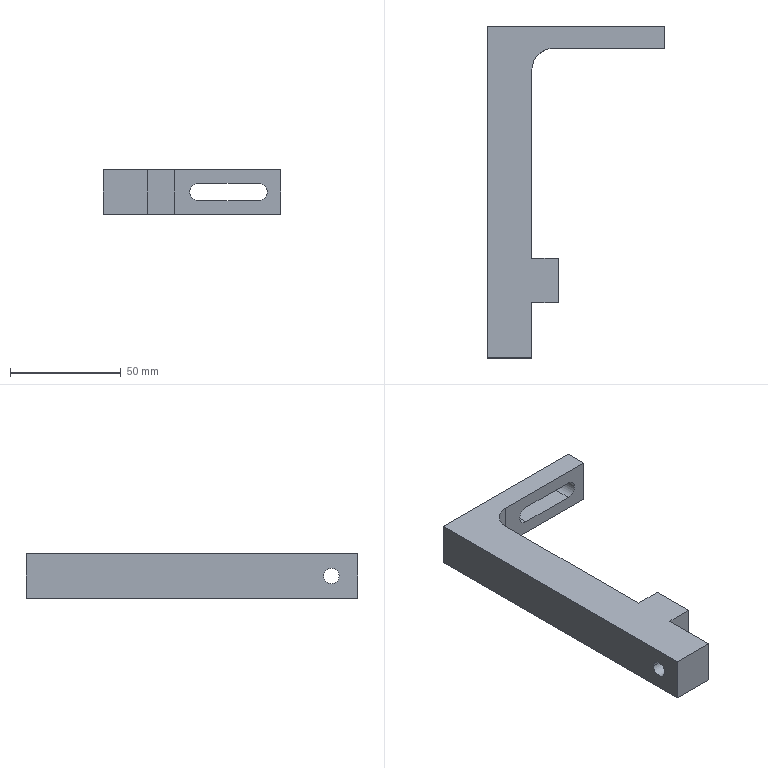Component | SolidWorks | GuideMechanism-1_LimitRollerSeat-1 | 1 solid | 19 faces | box 80 x 150 x 20 mm | volume 73797 mm3 | plane 14 | cylinder 5 | commonest cylinder face diameters 7 x2 8 x2 20 x1
build123d program:
from build123d import *

# Parameters (mm, degrees)
SKETCH1_W           = 80
SKETCH1_H           = 125
BOSS_EXTRUDE1_DEPTH = 20
SKETCH2_W           = 60
SKETCH2_H           = 95
CUT_EXTRUDE1_DEPTH  = 77.852
BOSS_EXTRUDE2_DEPTH = 20
SKETCH4_R           = 4
CUT_EXTRUDE2_DEPTH  = 157.525
CUT_EXTRUDE3_DEPTH  = 157.525
SKETCH6_R           = 3.5
CUT_EXTRUDE4_DEPTH  = 121.234
SKETCH7_W           = 48
SKETCH7_H           = 20
CUT_EXTRUDE5_DEPTH  = 99.266
FILLET1_R           = 10


with BuildPart() as part:
    # Sketch1 → Boss-Extrude1 (new body)
    with BuildSketch(Plane.XY):
        Rectangle(SKETCH1_W, SKETCH1_H)
    extrude(amount=BOSS_EXTRUDE1_DEPTH)

    # Sketch2 → Cut-Extrude1 (cut, through all)
    with BuildSketch(Plane.XY.offset(20)):
        with Locations((10, 5)):
            Rectangle(SKETCH2_W, SKETCH2_H)
    extrude(amount=-CUT_EXTRUDE1_DEPTH, mode=Mode.SUBTRACT)

    # Sketch3 → Boss-Extrude2 (add)
    with BuildSketch(Plane.XY.offset(20)):
        Polygon((-20, -42.5), (-20, -87.5), (-40, -87.5), (-40, -62.5), align=None)
    extrude(amount=-BOSS_EXTRUDE2_DEPTH)

    # Sketch4 → Cut-Extrude2 (cut, through all)
    with BuildSketch(Plane(origin=(0, 62.5, 0), x_dir=(1, 0, 0), z_dir=(0, 1, 0))):
        with Locations(Location((30, -10, 0), (0, 0, 270))):
            Circle(SKETCH4_R)
    extrude(amount=-CUT_EXTRUDE2_DEPTH, mode=Mode.SUBTRACT)

    # Sketch5 → Cut-Extrude3 (cut, through all)
    with BuildSketch(Plane(origin=(0, 62.5, 0), x_dir=(1, 0, 0), z_dir=(0, 1, 0))):
        with BuildLine():
            Line((30, -14), (3, -14))
            ThreePointArc((3, -14), (-1, -10), (3, -6))
            Line((3, -6), (30, -6))
            ThreePointArc((30, -6), (34, -10), (30, -14))
        make_face()
    extrude(amount=-CUT_EXTRUDE3_DEPTH, mode=Mode.SUBTRACT)

    # Sketch6 → Cut-Extrude4 (cut, through all)
    with BuildSketch(Plane.ZY.offset(40)):
        with Locations(Location((10, -75.5, 0), (0, 0, 270))):
            Circle(SKETCH6_R)
    extrude(amount=-CUT_EXTRUDE4_DEPTH, mode=Mode.SUBTRACT)

    # Sketch7 → Cut-Extrude5 (cut, through all)
    with BuildSketch(Plane.XY.offset(20)):
        with Locations((16, -52.5)):
            Rectangle(SKETCH7_W, SKETCH7_H)
    extrude(amount=-CUT_EXTRUDE5_DEPTH, mode=Mode.SUBTRACT)

    # Fillet1
    fillet1_edges = [part.edges().sort_by_distance(p)[0] for p in [
        (-20, 52.5, 10),
    ]]
    fillet(fillet1_edges, radius=FILLET1_R)


solid = part.part

# Placed as in the assembly
solid = solid.moved(Location((-505.272, -306.266, 1151.5), (0, 0, 0)))
STEP:
#1=COLOUR_RGB('',0.7922,0.8196,0.9333);
#2=FILL_AREA_STYLE_COLOUR('',#1);
#3=FILL_AREA_STYLE('',(#2));
#4=SURFACE_STYLE_FILL_AREA(#3);
#5=SURFACE_SIDE_STYLE('',(#4));
#6=SURFACE_STYLE_USAGE(.BOTH.,#5);
#7=PRESENTATION_STYLE_ASSIGNMENT((#6));
#8=CARTESIAN_POINT('',(-20.68,-15.168,45.728));
#9=VERTEX_POINT('',#8);
#10=CARTESIAN_POINT('',(-20.68,-14.892,45.728));
#11=VERTEX_POINT('',#10);
#12=CARTESIAN_POINT('',(-20.68,-15.03,45.728));
#13=DIRECTION('',(1.,0.,0.));
#14=DIRECTION('',(0.,1.,0.));
#15=AXIS2_PLACEMENT_3D('',#12,#13,#14);
#16=CIRCLE('',#15,0.1378);
#17=EDGE_CURVE('',#9,#11,#16,.T.);
#18=ORIENTED_EDGE('',*,*,#17,.T.);
#19=CARTESIAN_POINT('',(-21.467,-14.892,45.728));
#20=VERTEX_POINT('',#19);
#21=CARTESIAN_POINT('',(-18.318,-14.892,45.728));
#22=DIRECTION('',(-1.,-0.,0.));
#23=VECTOR('',#22,39.37);
#24=LINE('',#21,#23);
#25=EDGE_CURVE('',#11,#20,#24,.T.);
#26=ORIENTED_EDGE('',*,*,#25,.T.);
#27=CARTESIAN_POINT('',(-21.467,-15.168,45.728));
#28=VERTEX_POINT('',#27);
#29=CARTESIAN_POINT('',(-21.467,-15.03,45.728));
#30=DIRECTION('',(-1.,-0.,0.));
#31=DIRECTION('',(0.,-1.,0.));
#32=AXIS2_PLACEMENT_3D('',#29,#30,#31);
#33=CIRCLE('',#32,0.1378);
#34=EDGE_CURVE('',#20,#28,#33,.T.);
#35=ORIENTED_EDGE('',*,*,#34,.T.);
#36=CARTESIAN_POINT('',(-18.318,-15.168,45.728));
#37=DIRECTION('',(-1.,-0.,0.));
#38=VECTOR('',#37,39.37);
#39=LINE('',#36,#38);
#40=EDGE_CURVE('',#9,#28,#39,.T.);
#41=ORIENTED_EDGE('',*,*,#40,.F.);
#42=EDGE_LOOP('',(#18,#26,#35,#41));
#43=FACE_OUTER_BOUND('',#42,.T.);
#44=CARTESIAN_POINT('',(-18.318,-15.03,45.728));
#45=DIRECTION('',(-1.,-0.,0.));
#46=DIRECTION('',(0.,-1.,0.));
#47=AXIS2_PLACEMENT_3D('',#44,#45,#46);
#48=CYLINDRICAL_SURFACE('',#47,0.1378);
#49=ADVANCED_FACE('',(#43),#48,.F.);
#50=CARTESIAN_POINT('',(-18.711,-9.991,45.886));
#51=VERTEX_POINT('',#50);
#52=CARTESIAN_POINT('',(-18.711,-9.597,45.886));
#53=VERTEX_POINT('',#52);
#54=CARTESIAN_POINT('',(-18.711,-15.503,45.886));
#55=DIRECTION('',(0.,1.,0.));
#56=VECTOR('',#55,39.37);
#57=LINE('',#54,#56);
#58=EDGE_CURVE('',#51,#53,#57,.T.);
#59=ORIENTED_EDGE('',*,*,#58,.T.);
#60=CARTESIAN_POINT('',(-18.711,-9.597,45.571));
#61=VERTEX_POINT('',#60);
#62=CARTESIAN_POINT('',(-18.711,-9.597,45.728));
#63=DIRECTION('',(0.,1.,0.));
#64=DIRECTION('',(0.,0.,1.));
#65=AXIS2_PLACEMENT_3D('',#62,#63,#64);
#66=CIRCLE('',#65,0.1575);
#67=EDGE_CURVE('',#53,#61,#66,.T.);
#68=ORIENTED_EDGE('',*,*,#67,.T.);
#69=CARTESIAN_POINT('',(-18.711,-9.991,45.571));
#70=VERTEX_POINT('',#69);
#71=CARTESIAN_POINT('',(-18.711,-15.503,45.571));
#72=DIRECTION('',(0.,1.,0.));
#73=VECTOR('',#72,39.37);
#74=LINE('',#71,#73);
#75=EDGE_CURVE('',#70,#61,#74,.T.);
#76=ORIENTED_EDGE('',*,*,#75,.F.);
#77=CARTESIAN_POINT('',(-18.711,-9.991,45.728));
#78=DIRECTION('',(0.,1.,0.));
#79=DIRECTION('',(0.,0.,1.));
#80=AXIS2_PLACEMENT_3D('',#77,#78,#79);
#81=CIRCLE('',#80,0.1575);
#82=EDGE_CURVE('',#51,#70,#81,.T.);
#83=ORIENTED_EDGE('',*,*,#82,.F.);
#84=EDGE_LOOP('',(#59,#68,#76,#83));
#85=FACE_OUTER_BOUND('',#84,.T.);
#86=CARTESIAN_POINT('',(-18.711,-15.503,45.728));
#87=DIRECTION('',(0.,1.,0.));
#88=DIRECTION('',(0.,0.,1.));
#89=AXIS2_PLACEMENT_3D('',#86,#87,#88);
#90=CYLINDRICAL_SURFACE('',#89,0.1575);
#91=ADVANCED_FACE('',(#85),#90,.F.);
#92=CARTESIAN_POINT('',(-18.318,-9.991,46.122));
#93=VERTEX_POINT('',#92);
#94=CARTESIAN_POINT('',(-18.318,-9.597,46.122));
#95=VERTEX_POINT('',#94);
#96=CARTESIAN_POINT('',(-18.318,-9.597,46.122));
#97=DIRECTION('',(-0.,1.,0.));
#98=VECTOR('',#97,39.37);
#99=LINE('',#96,#98);
#100=EDGE_CURVE('',#93,#95,#99,.T.);
#101=ORIENTED_EDGE('',*,*,#100,.F.);
#102=CARTESIAN_POINT('',(-18.318,-9.991,45.335));
#103=VERTEX_POINT('',#102);
#104=CARTESIAN_POINT('',(-18.318,-9.991,45.335));
#105=DIRECTION('',(0.,0.,1.));
#106=VECTOR('',#105,39.37);
#107=LINE('',#104,#106);
#108=EDGE_CURVE('',#103,#93,#107,.T.);
#109=ORIENTED_EDGE('',*,*,#108,.F.);
#110=CARTESIAN_POINT('',(-18.318,-9.597,45.335));
#111=VERTEX_POINT('',#110);
#112=CARTESIAN_POINT('',(-18.318,-9.597,45.335));
#113=DIRECTION('',(-0.,1.,0.));
#114=VECTOR('',#113,39.37);
#115=LINE('',#112,#114);
#116=EDGE_CURVE('',#103,#111,#115,.T.);
#117=ORIENTED_EDGE('',*,*,#116,.T.);
#118=CARTESIAN_POINT('',(-18.318,-9.597,46.122));
#119=DIRECTION('',(0.,0.,-1.));
#120=VECTOR('',#119,39.37);
#121=LINE('',#118,#120);
#122=EDGE_CURVE('',#95,#111,#121,.T.);
#123=ORIENTED_EDGE('',*,*,#122,.F.);
#124=EDGE_LOOP('',(#101,#109,#117,#123));
#125=FACE_OUTER_BOUND('',#124,.T.);
#126=CARTESIAN_POINT('',(-18.318,-9.597,46.122));
#127=DIRECTION('',(-1.,-0.,0.));
#128=DIRECTION('',(0.,-1.,0.));
#129=AXIS2_PLACEMENT_3D('',#126,#127,#128);
#130=PLANE('',#129);
#131=ADVANCED_FACE('',(#125),#130,.F.);
#132=ORIENTED_EDGE('',*,*,#67,.F.);
#133=CARTESIAN_POINT('',(-19.774,-9.597,45.886));
#134=VERTEX_POINT('',#133);
#135=CARTESIAN_POINT('',(-18.711,-9.597,45.886));
#136=DIRECTION('',(1.,0.,-0.));
#137=VECTOR('',#136,39.37);
#138=LINE('',#135,#137);
#139=EDGE_CURVE('',#134,#53,#138,.T.);
#140=ORIENTED_EDGE('',*,*,#139,.F.);
#141=CARTESIAN_POINT('',(-19.774,-9.597,45.571));
#142=VERTEX_POINT('',#141);
#143=CARTESIAN_POINT('',(-19.774,-9.597,45.728));
#144=DIRECTION('',(0.,1.,0.));
#145=DIRECTION('',(0.,0.,1.));
#146=AXIS2_PLACEMENT_3D('',#143,#144,#145);
#147=CIRCLE('',#146,0.1575);
#148=EDGE_CURVE('',#142,#134,#147,.T.);
#149=ORIENTED_EDGE('',*,*,#148,.F.);
#150=CARTESIAN_POINT('',(-18.711,-9.597,45.571));
#151=DIRECTION('',(-1.,0.,0.));
#152=VECTOR('',#151,39.37);
#153=LINE('',#150,#152);
#154=EDGE_CURVE('',#61,#142,#153,.T.);
#155=ORIENTED_EDGE('',*,*,#154,.F.);
#156=EDGE_LOOP('',(#132,#140,#149,#155));
#157=FACE_BOUND('',#156,.T.);
#158=CARTESIAN_POINT('',(-21.467,-9.597,45.335));
#159=VERTEX_POINT('',#158);
#160=CARTESIAN_POINT('',(-21.467,-9.597,45.335));
#161=DIRECTION('',(-1.,0.,0.));
#162=VECTOR('',#161,39.37);
#163=LINE('',#160,#162);
#164=EDGE_CURVE('',#111,#159,#163,.T.);
#165=ORIENTED_EDGE('',*,*,#164,.T.);
#166=CARTESIAN_POINT('',(-21.467,-9.597,46.122));
#167=VERTEX_POINT('',#166);
#168=CARTESIAN_POINT('',(-21.467,-9.597,46.122));
#169=DIRECTION('',(0.,0.,-1.));
#170=VECTOR('',#169,39.37);
#171=LINE('',#168,#170);
#172=EDGE_CURVE('',#167,#159,#171,.T.);
#173=ORIENTED_EDGE('',*,*,#172,.F.);
#174=CARTESIAN_POINT('',(-21.467,-9.597,46.122));
#175=DIRECTION('',(-1.,0.,0.));
#176=VECTOR('',#175,39.37);
#177=LINE('',#174,#176);
#178=EDGE_CURVE('',#95,#167,#177,.T.);
#179=ORIENTED_EDGE('',*,*,#178,.F.);
#180=ORIENTED_EDGE('',*,*,#122,.T.);
#181=EDGE_LOOP('',(#165,#173,#179,#180));
#182=FACE_OUTER_BOUND('',#181,.T.);
#183=CARTESIAN_POINT('',(-21.467,-9.597,46.122));
#184=DIRECTION('',(0.,-1.,0.));
#185=DIRECTION('',(0.,0.,-1.));
#186=AXIS2_PLACEMENT_3D('',#183,#184,#185);
#187=PLANE('',#186);
#188=ADVANCED_FACE('',(#157,#182),#187,.F.);
#189=CARTESIAN_POINT('',(-21.467,-15.03,45.728));
#190=DIRECTION('',(-1.,-0.,0.));
#191=DIRECTION('',(0.,-1.,0.));
#192=AXIS2_PLACEMENT_3D('',#189,#190,#191);
#193=CIRCLE('',#192,0.1378);
#194=EDGE_CURVE('',#28,#20,#193,.T.);
#195=ORIENTED_EDGE('',*,*,#194,.F.);
#196=ORIENTED_EDGE('',*,*,#34,.F.);
#197=EDGE_LOOP('',(#195,#196));
#198=FACE_BOUND('',#197,.T.);
#199=CARTESIAN_POINT('',(-21.467,-15.503,45.335));
#200=VERTEX_POINT('',#199);
#201=CARTESIAN_POINT('',(-21.467,-9.597,45.335));
#202=DIRECTION('',(0.,-1.,0.));
#203=VECTOR('',#202,39.37);
#204=LINE('',#201,#203);
#205=EDGE_CURVE('',#159,#200,#204,.T.);
#206=ORIENTED_EDGE('',*,*,#205,.T.);
#207=CARTESIAN_POINT('',(-21.467,-15.503,46.122));
#208=VERTEX_POINT('',#207);
#209=CARTESIAN_POINT('',(-21.467,-15.503,45.335));
#210=DIRECTION('',(0.,0.,1.));
#211=VECTOR('',#210,39.37);
#212=LINE('',#209,#211);
#213=EDGE_CURVE('',#200,#208,#212,.T.);
#214=ORIENTED_EDGE('',*,*,#213,.T.);
#215=CARTESIAN_POINT('',(-21.467,-9.597,46.122));
#216=DIRECTION('',(0.,-1.,0.));
#217=VECTOR('',#216,39.37);
#218=LINE('',#215,#217);
#219=EDGE_CURVE('',#167,#208,#218,.T.);
#220=ORIENTED_EDGE('',*,*,#219,.F.);
#221=ORIENTED_EDGE('',*,*,#172,.T.);
#222=EDGE_LOOP('',(#206,#214,#220,#221));
#223=FACE_OUTER_BOUND('',#222,.T.);
#224=CARTESIAN_POINT('',(-21.467,-9.597,46.122));
#225=DIRECTION('',(1.,0.,0.));
#226=DIRECTION('',(-0.,1.,0.));
#227=AXIS2_PLACEMENT_3D('',#224,#225,#226);
#228=PLANE('',#227);
#229=ADVANCED_FACE('',(#198,#223),#228,.F.);
#230=CARTESIAN_POINT('',(-20.68,-14.518,45.335));
#231=VERTEX_POINT('',#230);
#232=CARTESIAN_POINT('',(-20.208,-14.518,45.335));
#233=VERTEX_POINT('',#232);
#234=CARTESIAN_POINT('',(-21.467,-14.518,45.335));
#235=DIRECTION('',(1.,0.,0.));
#236=VECTOR('',#235,39.37);
#237=LINE('',#234,#236);
#238=EDGE_CURVE('',#231,#233,#237,.T.);
#239=ORIENTED_EDGE('',*,*,#238,.T.);
#240=CARTESIAN_POINT('',(-20.208,-14.518,46.122));
#241=VERTEX_POINT('',#240);
#242=CARTESIAN_POINT('',(-20.208,-14.518,45.335));
#243=DIRECTION('',(0.,0.,1.));
#244=VECTOR('',#243,39.37);
#245=LINE('',#242,#244);
#246=EDGE_CURVE('',#233,#241,#245,.T.);
#247=ORIENTED_EDGE('',*,*,#246,.T.);
#248=CARTESIAN_POINT('',(-20.68,-14.518,46.122));
#249=VERTEX_POINT('',#248);
#250=CARTESIAN_POINT('',(-21.467,-14.518,46.122));
#251=DIRECTION('',(1.,0.,0.));
#252=VECTOR('',#251,39.37);
#253=LINE('',#250,#252);
#254=EDGE_CURVE('',#249,#241,#253,.T.);
#255=ORIENTED_EDGE('',*,*,#254,.F.);
#256=CARTESIAN_POINT('',(-20.68,-14.518,46.122));
#257=DIRECTION('',(0.,0.,-1.));
#258=VECTOR('',#257,39.37);
#259=LINE('',#256,#258);
#260=EDGE_CURVE('',#249,#231,#259,.T.);
#261=ORIENTED_EDGE('',*,*,#260,.T.);
#262=EDGE_LOOP('',(#239,#247,#255,#261));
#263=FACE_OUTER_BOUND('',#262,.T.);
#264=CARTESIAN_POINT('',(-21.467,-14.518,46.122));
#265=DIRECTION('',(0.,1.,0.));
#266=DIRECTION('',(0.,0.,1.));
#267=AXIS2_PLACEMENT_3D('',#264,#265,#266);
#268=PLANE('',#267);
#269=ADVANCED_FACE('',(#263),#268,.F.);
#270=CARTESIAN_POINT('',(-20.208,-13.731,46.122));
#271=VERTEX_POINT('',#270);
#272=CARTESIAN_POINT('',(-20.208,-13.731,46.122));
#273=DIRECTION('',(0.,-1.,0.));
#274=VECTOR('',#273,39.37);
#275=LINE('',#272,#274);
#276=EDGE_CURVE('',#271,#241,#275,.T.);
#277=ORIENTED_EDGE('',*,*,#276,.F.);
#278=CARTESIAN_POINT('',(-20.68,-13.731,46.122));
#279=VERTEX_POINT('',#278);
#280=CARTESIAN_POINT('',(-18.318,-13.731,46.122));
#281=DIRECTION('',(1.,0.,0.));
#282=VECTOR('',#281,39.37);
#283=LINE('',#280,#282);
#284=EDGE_CURVE('',#279,#271,#283,.T.);
#285=ORIENTED_EDGE('',*,*,#284,.F.);
#286=CARTESIAN_POINT('',(-20.68,-10.384,46.122));
#287=VERTEX_POINT('',#286);
#288=CARTESIAN_POINT('',(-20.68,-9.991,46.122));
#289=DIRECTION('',(0.,-1.,0.));
#290=VECTOR('',#289,39.37);
#291=LINE('',#288,#290);
#292=EDGE_CURVE('',#287,#279,#291,.T.);
#293=ORIENTED_EDGE('',*,*,#292,.F.);
#294=CARTESIAN_POINT('',(-20.286,-9.991,46.122));
#295=VERTEX_POINT('',#294);
#296=CARTESIAN_POINT('',(-20.286,-10.384,46.122));
#297=DIRECTION('',(0.,0.,-1.));
#298=DIRECTION('',(1.,0.,0.));
#299=AXIS2_PLACEMENT_3D('',#296,#297,#298);
#300=CIRCLE('',#299,0.3937);
#301=EDGE_CURVE('',#287,#295,#300,.T.);
#302=ORIENTED_EDGE('',*,*,#301,.T.);
#303=CARTESIAN_POINT('',(-18.318,-9.991,46.122));
#304=DIRECTION('',(-1.,0.,0.));
#305=VECTOR('',#304,39.37);
#306=LINE('',#303,#305);
#307=EDGE_CURVE('',#93,#295,#306,.T.);
#308=ORIENTED_EDGE('',*,*,#307,.F.);
#309=ORIENTED_EDGE('',*,*,#100,.T.);
#310=ORIENTED_EDGE('',*,*,#178,.T.);
#311=ORIENTED_EDGE('',*,*,#219,.T.);
#312=CARTESIAN_POINT('',(-20.68,-15.503,46.122));
#313=VERTEX_POINT('',#312);
#314=CARTESIAN_POINT('',(-20.68,-15.503,46.122));
#315=DIRECTION('',(1.,0.,0.));
#316=VECTOR('',#315,39.37);
#317=LINE('',#314,#316);
#318=EDGE_CURVE('',#208,#313,#317,.T.);
#319=ORIENTED_EDGE('',*,*,#318,.T.);
#320=CARTESIAN_POINT('',(-20.68,-13.731,46.122));
#321=DIRECTION('',(-0.,1.,0.));
#322=VECTOR('',#321,39.37);
#323=LINE('',#320,#322);
#324=EDGE_CURVE('',#313,#249,#323,.T.);
#325=ORIENTED_EDGE('',*,*,#324,.T.);
#326=ORIENTED_EDGE('',*,*,#254,.T.);
#327=EDGE_LOOP('',(#277,#285,#293,#302,#308,#309,#310,#311,#319,#325,#326));
#328=FACE_OUTER_BOUND('',#327,.T.);
#329=CARTESIAN_POINT('',(-19.893,-12.058,46.122));
#330=DIRECTION('',(0.,0.,1.));
#331=DIRECTION('',(1.,0.,0.));
#332=AXIS2_PLACEMENT_3D('',#329,#330,#331);
#333=PLANE('',#332);
#334=ADVANCED_FACE('',(#328),#333,.T.);
#335=CARTESIAN_POINT('',(-20.68,-13.731,45.335));
#336=VERTEX_POINT('',#335);
#337=CARTESIAN_POINT('',(-20.208,-13.731,45.335));
#338=VERTEX_POINT('',#337);
#339=CARTESIAN_POINT('',(-18.318,-13.731,45.335));
#340=DIRECTION('',(1.,0.,0.));
#341=VECTOR('',#340,39.37);
#342=LINE('',#339,#341);
#343=EDGE_CURVE('',#336,#338,#342,.T.);
#344=ORIENTED_EDGE('',*,*,#343,.T.);
#345=CARTESIAN_POINT('',(-20.208,-13.731,45.335));
#346=DIRECTION('',(0.,-1.,0.));
#347=VECTOR('',#346,39.37);
#348=LINE('',#345,#347);
#349=EDGE_CURVE('',#338,#233,#348,.T.);
#350=ORIENTED_EDGE('',*,*,#349,.T.);
#351=ORIENTED_EDGE('',*,*,#238,.F.);
#352=CARTESIAN_POINT('',(-20.68,-15.503,45.335));
#353=VERTEX_POINT('',#352);
#354=CARTESIAN_POINT('',(-20.68,-13.731,45.335));
#355=DIRECTION('',(-0.,1.,0.));
#356=VECTOR('',#355,39.37);
#357=LINE('',#354,#356);
#358=EDGE_CURVE('',#353,#231,#357,.T.);
#359=ORIENTED_EDGE('',*,*,#358,.F.);
#360=CARTESIAN_POINT('',(-20.68,-15.503,45.335));
#361=DIRECTION('',(1.,0.,0.));
#362=VECTOR('',#361,39.37);
#363=LINE('',#360,#362);
#364=EDGE_CURVE('',#200,#353,#363,.T.);
#365=ORIENTED_EDGE('',*,*,#364,.F.);
#366=ORIENTED_EDGE('',*,*,#205,.F.);
#367=ORIENTED_EDGE('',*,*,#164,.F.);
#368=ORIENTED_EDGE('',*,*,#116,.F.);
#369=CARTESIAN_POINT('',(-20.286,-9.991,45.335));
#370=VERTEX_POINT('',#369);
#371=CARTESIAN_POINT('',(-18.318,-9.991,45.335));
#372=DIRECTION('',(-1.,0.,0.));
#373=VECTOR('',#372,39.37);
#374=LINE('',#371,#373);
#375=EDGE_CURVE('',#103,#370,#374,.T.);
#376=ORIENTED_EDGE('',*,*,#375,.T.);
#377=CARTESIAN_POINT('',(-20.68,-10.384,45.335));
#378=VERTEX_POINT('',#377);
#379=CARTESIAN_POINT('',(-20.286,-10.384,45.335));
#380=DIRECTION('',(0.,0.,1.));
#381=DIRECTION('',(1.,0.,0.));
#382=AXIS2_PLACEMENT_3D('',#379,#380,#381);
#383=CIRCLE('',#382,0.3937);
#384=EDGE_CURVE('',#370,#378,#383,.T.);
#385=ORIENTED_EDGE('',*,*,#384,.T.);
#386=CARTESIAN_POINT('',(-20.68,-9.991,45.335));
#387=DIRECTION('',(0.,-1.,0.));
#388=VECTOR('',#387,39.37);
#389=LINE('',#386,#388);
#390=EDGE_CURVE('',#378,#336,#389,.T.);
#391=ORIENTED_EDGE('',*,*,#390,.T.);
#392=EDGE_LOOP('',(#344,#350,#351,#359,#365,#366,#367,#368,#376,#385,#391));
#393=FACE_OUTER_BOUND('',#392,.T.);
#394=CARTESIAN_POINT('',(-19.893,-12.058,45.335));
#395=DIRECTION('',(0.,0.,1.));
#396=DIRECTION('',(1.,0.,0.));
#397=AXIS2_PLACEMENT_3D('',#394,#395,#396);
#398=PLANE('',#397);
#399=ADVANCED_FACE('',(#393),#398,.F.);
#400=ORIENTED_EDGE('',*,*,#284,.T.);
#401=CARTESIAN_POINT('',(-20.208,-13.731,45.335));
#402=DIRECTION('',(0.,0.,1.));
#403=VECTOR('',#402,39.37);
#404=LINE('',#401,#403);
#405=EDGE_CURVE('',#338,#271,#404,.T.);
#406=ORIENTED_EDGE('',*,*,#405,.F.);
#407=ORIENTED_EDGE('',*,*,#343,.F.);
#408=CARTESIAN_POINT('',(-20.68,-13.731,45.335));
#409=DIRECTION('',(0.,0.,1.));
#410=VECTOR('',#409,39.37);
#411=LINE('',#408,#410);
#412=EDGE_CURVE('',#336,#279,#411,.T.);
#413=ORIENTED_EDGE('',*,*,#412,.T.);
#414=EDGE_LOOP('',(#400,#406,#407,#413));
#415=FACE_OUTER_BOUND('',#414,.T.);
#416=CARTESIAN_POINT('',(-18.318,-13.731,45.335));
#417=DIRECTION('',(0.,-1.,0.));
#418=DIRECTION('',(1.,0.,0.));
#419=AXIS2_PLACEMENT_3D('',#416,#417,#418);
#420=PLANE('',#419);
#421=ADVANCED_FACE('',(#415),#420,.F.);
#422=ORIENTED_EDGE('',*,*,#390,.F.);
#423=CARTESIAN_POINT('',(-20.68,-10.384,46.122));
#424=DIRECTION('',(0.,0.,1.));
#425=VECTOR('',#424,39.37);
#426=LINE('',#423,#425);
#427=EDGE_CURVE('',#378,#287,#426,.T.);
#428=ORIENTED_EDGE('',*,*,#427,.T.);
#429=ORIENTED_EDGE('',*,*,#292,.T.);
#430=ORIENTED_EDGE('',*,*,#412,.F.);
#431=EDGE_LOOP('',(#422,#428,#429,#430));
#432=FACE_OUTER_BOUND('',#431,.T.);
#433=CARTESIAN_POINT('',(-20.68,-9.991,45.335));
#434=DIRECTION('',(-1.,-0.,0.));
#435=DIRECTION('',(0.,-1.,0.));
#436=AXIS2_PLACEMENT_3D('',#433,#434,#435);
#437=PLANE('',#436);
#438=ADVANCED_FACE('',(#432),#437,.F.);
#439=CARTESIAN_POINT('',(-19.774,-9.991,45.571));
#440=VERTEX_POINT('',#439);
#441=CARTESIAN_POINT('',(-19.774,-9.991,45.886));
#442=VERTEX_POINT('',#441);
#443=CARTESIAN_POINT('',(-19.774,-9.991,45.728));
#444=DIRECTION('',(0.,1.,0.));
#445=DIRECTION('',(0.,0.,1.));
#446=AXIS2_PLACEMENT_3D('',#443,#444,#445);
#447=CIRCLE('',#446,0.1575);
#448=EDGE_CURVE('',#440,#442,#447,.T.);
#449=ORIENTED_EDGE('',*,*,#448,.T.);
#450=CARTESIAN_POINT('',(-18.318,-9.991,45.886));
#451=DIRECTION('',(1.,0.,-0.));
#452=VECTOR('',#451,39.37);
#453=LINE('',#450,#452);
#454=EDGE_CURVE('',#442,#51,#453,.T.);
#455=ORIENTED_EDGE('',*,*,#454,.T.);
#456=ORIENTED_EDGE('',*,*,#82,.T.);
#457=CARTESIAN_POINT('',(-18.318,-9.991,45.571));
#458=DIRECTION('',(-1.,0.,0.));
#459=VECTOR('',#458,39.37);
#460=LINE('',#457,#459);
#461=EDGE_CURVE('',#70,#440,#460,.T.);
#462=ORIENTED_EDGE('',*,*,#461,.T.);
#463=EDGE_LOOP('',(#449,#455,#456,#462));
#464=FACE_BOUND('',#463,.T.);
#465=ORIENTED_EDGE('',*,*,#307,.T.);
#466=CARTESIAN_POINT('',(-20.286,-9.991,45.335));
#467=DIRECTION('',(0.,0.,-1.));
#468=VECTOR('',#467,39.37);
#469=LINE('',#466,#468);
#470=EDGE_CURVE('',#295,#370,#469,.T.);
#471=ORIENTED_EDGE('',*,*,#470,.T.);
#472=ORIENTED_EDGE('',*,*,#375,.F.);
#473=ORIENTED_EDGE('',*,*,#108,.T.);
#474=EDGE_LOOP('',(#465,#471,#472,#473));
#475=FACE_OUTER_BOUND('',#474,.T.);
#476=CARTESIAN_POINT('',(-18.318,-9.991,45.335));
#477=DIRECTION('',(0.,1.,0.));
#478=DIRECTION('',(0.,0.,1.));
#479=AXIS2_PLACEMENT_3D('',#476,#477,#478);
#480=PLANE('',#479);
#481=ADVANCED_FACE('',(#464,#475),#480,.F.);
#482=ORIENTED_EDGE('',*,*,#17,.F.);
#483=CARTESIAN_POINT('',(-20.68,-15.03,45.728));
#484=DIRECTION('',(1.,0.,0.));
#485=DIRECTION('',(0.,1.,0.));
#486=AXIS2_PLACEMENT_3D('',#483,#484,#485);
#487=CIRCLE('',#486,0.1378);
#488=EDGE_CURVE('',#11,#9,#487,.T.);
#489=ORIENTED_EDGE('',*,*,#488,.F.);
#490=EDGE_LOOP('',(#482,#489));
#491=FACE_BOUND('',#490,.T.);
#492=ORIENTED_EDGE('',*,*,#260,.F.);
#493=ORIENTED_EDGE('',*,*,#324,.F.);
#494=CARTESIAN_POINT('',(-20.68,-15.503,45.335));
#495=DIRECTION('',(0.,0.,1.));
#496=VECTOR('',#495,39.37);
#497=LINE('',#494,#496);
#498=EDGE_CURVE('',#353,#313,#497,.T.);
#499=ORIENTED_EDGE('',*,*,#498,.F.);
#500=ORIENTED_EDGE('',*,*,#358,.T.);
#501=EDGE_LOOP('',(#492,#493,#499,#500));
#502=FACE_OUTER_BOUND('',#501,.T.);
#503=CARTESIAN_POINT('',(-20.68,-13.731,45.335));
#504=DIRECTION('',(1.,0.,0.));
#505=DIRECTION('',(-0.,1.,0.));
#506=AXIS2_PLACEMENT_3D('',#503,#504,#505);
#507=PLANE('',#506);
#508=ADVANCED_FACE('',(#491,#502),#507,.T.);
#509=ORIENTED_EDGE('',*,*,#318,.F.);
#510=ORIENTED_EDGE('',*,*,#213,.F.);
#511=ORIENTED_EDGE('',*,*,#364,.T.);
#512=ORIENTED_EDGE('',*,*,#498,.T.);
#513=EDGE_LOOP('',(#509,#510,#511,#512));
#514=FACE_OUTER_BOUND('',#513,.T.);
#515=CARTESIAN_POINT('',(-20.68,-15.503,45.335));
#516=DIRECTION('',(0.,-1.,0.));
#517=DIRECTION('',(0.,0.,-1.));
#518=AXIS2_PLACEMENT_3D('',#515,#516,#517);
#519=PLANE('',#518);
#520=ADVANCED_FACE('',(#514),#519,.T.);
#521=CARTESIAN_POINT('',(-19.774,-15.503,45.571));
#522=DIRECTION('',(0.,1.,0.));
#523=VECTOR('',#522,39.37);
#524=LINE('',#521,#523);
#525=EDGE_CURVE('',#440,#142,#524,.T.);
#526=ORIENTED_EDGE('',*,*,#525,.T.);
#527=ORIENTED_EDGE('',*,*,#148,.T.);
#528=CARTESIAN_POINT('',(-19.774,-15.503,45.886));
#529=DIRECTION('',(0.,1.,0.));
#530=VECTOR('',#529,39.37);
#531=LINE('',#528,#530);
#532=EDGE_CURVE('',#442,#134,#531,.T.);
#533=ORIENTED_EDGE('',*,*,#532,.F.);
#534=ORIENTED_EDGE('',*,*,#448,.F.);
#535=EDGE_LOOP('',(#526,#527,#533,#534));
#536=FACE_OUTER_BOUND('',#535,.T.);
#537=CARTESIAN_POINT('',(-19.774,-15.503,45.728));
#538=DIRECTION('',(0.,1.,0.));
#539=DIRECTION('',(0.,0.,1.));
#540=AXIS2_PLACEMENT_3D('',#537,#538,#539);
#541=CYLINDRICAL_SURFACE('',#540,0.1575);
#542=ADVANCED_FACE('',(#536),#541,.F.);
#543=ORIENTED_EDGE('',*,*,#532,.T.);
#544=ORIENTED_EDGE('',*,*,#139,.T.);
#545=ORIENTED_EDGE('',*,*,#58,.F.);
#546=ORIENTED_EDGE('',*,*,#454,.F.);
#547=EDGE_LOOP('',(#543,#544,#545,#546));
#548=FACE_OUTER_BOUND('',#547,.T.);
#549=CARTESIAN_POINT('',(-18.711,-15.503,45.886));
#550=DIRECTION('',(0.,0.,1.));
#551=DIRECTION('',(1.,0.,-0.));
#552=AXIS2_PLACEMENT_3D('',#549,#550,#551);
#553=PLANE('',#552);
#554=ADVANCED_FACE('',(#548),#553,.F.);
#555=ORIENTED_EDGE('',*,*,#75,.T.);
#556=ORIENTED_EDGE('',*,*,#154,.T.);
#557=ORIENTED_EDGE('',*,*,#525,.F.);
#558=ORIENTED_EDGE('',*,*,#461,.F.);
#559=EDGE_LOOP('',(#555,#556,#557,#558));
#560=FACE_OUTER_BOUND('',#559,.T.);
#561=CARTESIAN_POINT('',(-18.711,-15.503,45.571));
#562=DIRECTION('',(-0.,0.,-1.));
#563=DIRECTION('',(-1.,0.,0.));
#564=AXIS2_PLACEMENT_3D('',#561,#562,#563);
#565=PLANE('',#564);
#566=ADVANCED_FACE('',(#560),#565,.F.);
#567=ORIENTED_EDGE('',*,*,#25,.F.);
#568=ORIENTED_EDGE('',*,*,#488,.T.);
#569=ORIENTED_EDGE('',*,*,#40,.T.);
#570=ORIENTED_EDGE('',*,*,#194,.T.);
#571=EDGE_LOOP('',(#567,#568,#569,#570));
#572=FACE_OUTER_BOUND('',#571,.T.);
#573=CARTESIAN_POINT('',(-18.318,-15.03,45.728));
#574=DIRECTION('',(-1.,-0.,0.));
#575=DIRECTION('',(0.,-1.,0.));
#576=AXIS2_PLACEMENT_3D('',#573,#574,#575);
#577=CYLINDRICAL_SURFACE('',#576,0.1378);
#578=ADVANCED_FACE('',(#572),#577,.F.);
#579=ORIENTED_EDGE('',*,*,#276,.T.);
#580=ORIENTED_EDGE('',*,*,#246,.F.);
#581=ORIENTED_EDGE('',*,*,#349,.F.);
#582=ORIENTED_EDGE('',*,*,#405,.T.);
#583=EDGE_LOOP('',(#579,#580,#581,#582));
#584=FACE_OUTER_BOUND('',#583,.T.);
#585=CARTESIAN_POINT('',(-20.208,-13.731,45.335));
#586=DIRECTION('',(-1.,-0.,0.));
#587=DIRECTION('',(0.,-1.,0.));
#588=AXIS2_PLACEMENT_3D('',#585,#586,#587);
#589=PLANE('',#588);
#590=ADVANCED_FACE('',(#584),#589,.F.);
#591=ORIENTED_EDGE('',*,*,#384,.F.);
#592=ORIENTED_EDGE('',*,*,#470,.F.);
#593=ORIENTED_EDGE('',*,*,#301,.F.);
#594=ORIENTED_EDGE('',*,*,#427,.F.);
#595=EDGE_LOOP('',(#591,#592,#593,#594));
#596=FACE_OUTER_BOUND('',#595,.T.);
#597=CARTESIAN_POINT('',(-20.286,-10.384,45.335));
#598=DIRECTION('',(0.,0.,-1.));
#599=DIRECTION('',(-1.,0.,0.));
#600=AXIS2_PLACEMENT_3D('',#597,#598,#599);
#601=CYLINDRICAL_SURFACE('',#600,0.3937);
#602=ADVANCED_FACE('',(#596),#601,.F.);
#603=CLOSED_SHELL('',(#49,#91,#131,#188,#229,#269,#334,#399,#421,#438,#481,#508,#520,#542,#554,#566,#578,#590,#602));
#604=MANIFOLD_SOLID_BREP('',#603);
#605=STYLED_ITEM('',(#7),#604);
#606=PRESENTATION_LAYER_ASSIGNMENT('','',(#605));
#607=CARTESIAN_POINT('',(0.,0.,0.));
#608=DIRECTION('',(0.,0.,1.));
#609=DIRECTION('',(1.,0.,0.));
#610=AXIS2_PLACEMENT_3D('',#607,#608,#609);
#611=(LENGTH_UNIT()NAMED_UNIT(*)SI_UNIT($,.METRE.));
#612=LENGTH_MEASURE_WITH_UNIT(LENGTH_MEASURE(0.0254),#611);
#613=DIMENSIONAL_EXPONENTS(1.,0.,0.,0.,0.,0.,0.);
#614=(CONVERSION_BASED_UNIT('',#612)LENGTH_UNIT()NAMED_UNIT(#613));
#615=UNCERTAINTY_MEASURE_WITH_UNIT(LENGTH_MEASURE(0.00001),#614,'','');
#616=(NAMED_UNIT(*)PLANE_ANGLE_UNIT()SI_UNIT($,.RADIAN.));
#617=(NAMED_UNIT(*)SI_UNIT($,.STERADIAN.)SOLID_ANGLE_UNIT());
#618=(GEOMETRIC_REPRESENTATION_CONTEXT(3)GLOBAL_UNCERTAINTY_ASSIGNED_CONTEXT((#615))GLOBAL_UNIT_ASSIGNED_CONTEXT((#614,#616,#617))REPRESENTATION_CONTEXT('',''));
#619=ADVANCED_BREP_SHAPE_REPRESENTATION('',(#604,#610),#618);
#620=(LENGTH_UNIT()NAMED_UNIT(*)SI_UNIT($,.METRE.));
#621=LENGTH_MEASURE_WITH_UNIT(LENGTH_MEASURE(0.0254),#620);
#622=DIMENSIONAL_EXPONENTS(1.,0.,0.,0.,0.,0.,0.);
#623=(CONVERSION_BASED_UNIT('',#621)LENGTH_UNIT()NAMED_UNIT(#622));
#624=UNCERTAINTY_MEASURE_WITH_UNIT(LENGTH_MEASURE(0.00001),#623,'','');
#625=(NAMED_UNIT(*)PLANE_ANGLE_UNIT()SI_UNIT($,.RADIAN.));
#626=(NAMED_UNIT(*)SI_UNIT($,.STERADIAN.)SOLID_ANGLE_UNIT());
#627=(GEOMETRIC_REPRESENTATION_CONTEXT(3)GLOBAL_UNCERTAINTY_ASSIGNED_CONTEXT((#624))GLOBAL_UNIT_ASSIGNED_CONTEXT((#623,#625,#626))REPRESENTATION_CONTEXT('',''));
#628=MECHANICAL_DESIGN_GEOMETRIC_PRESENTATION_REPRESENTATION('',(#605),#627);